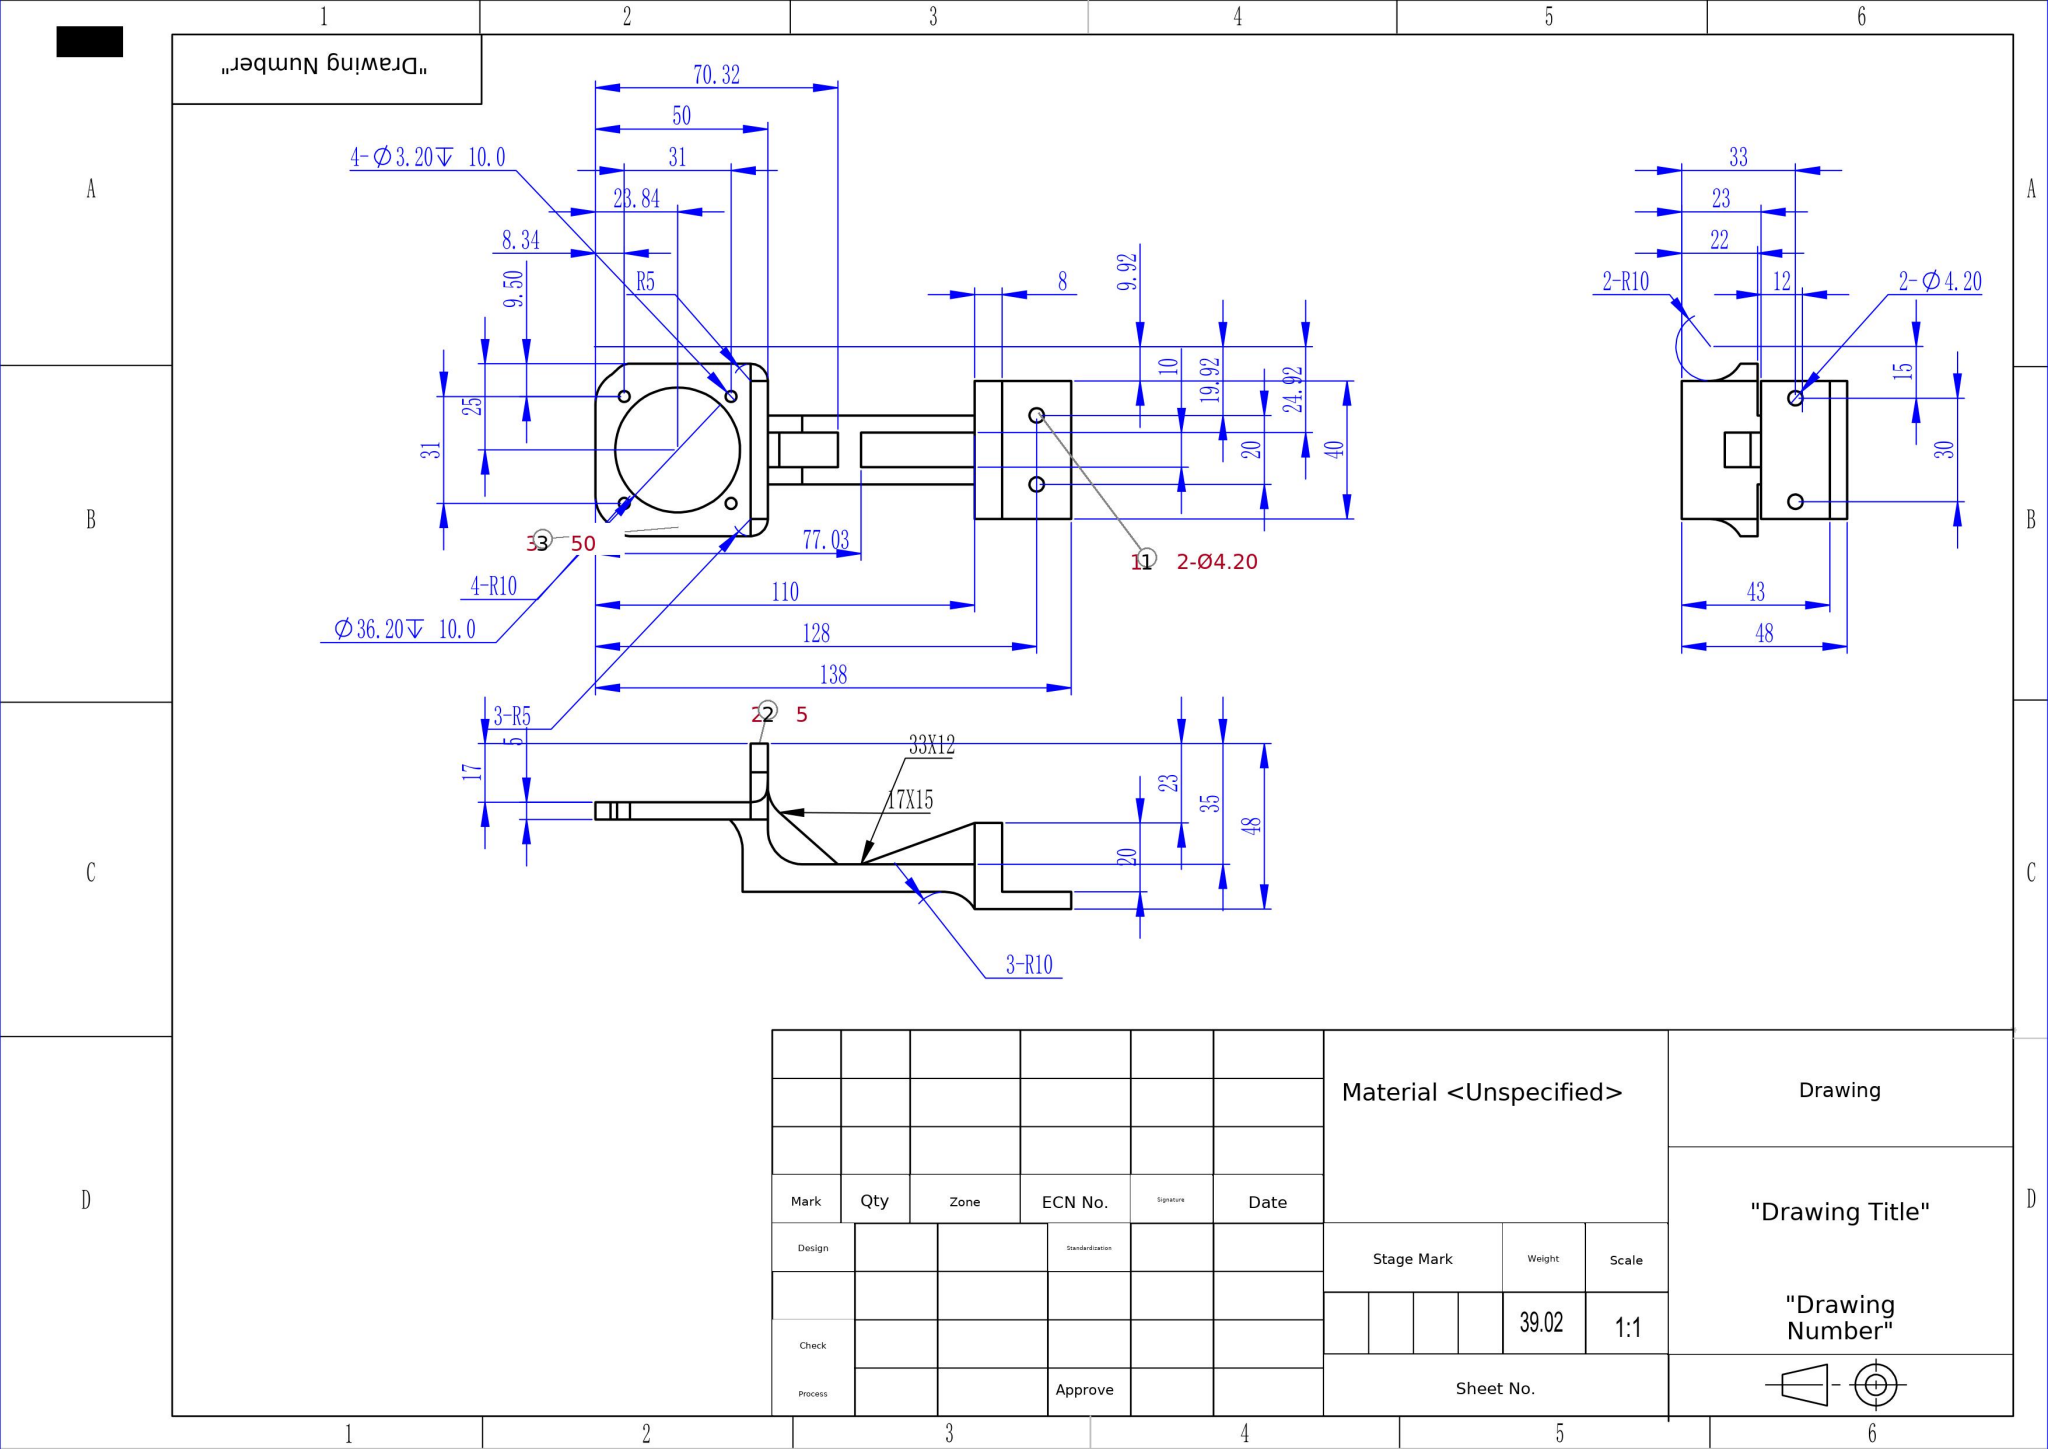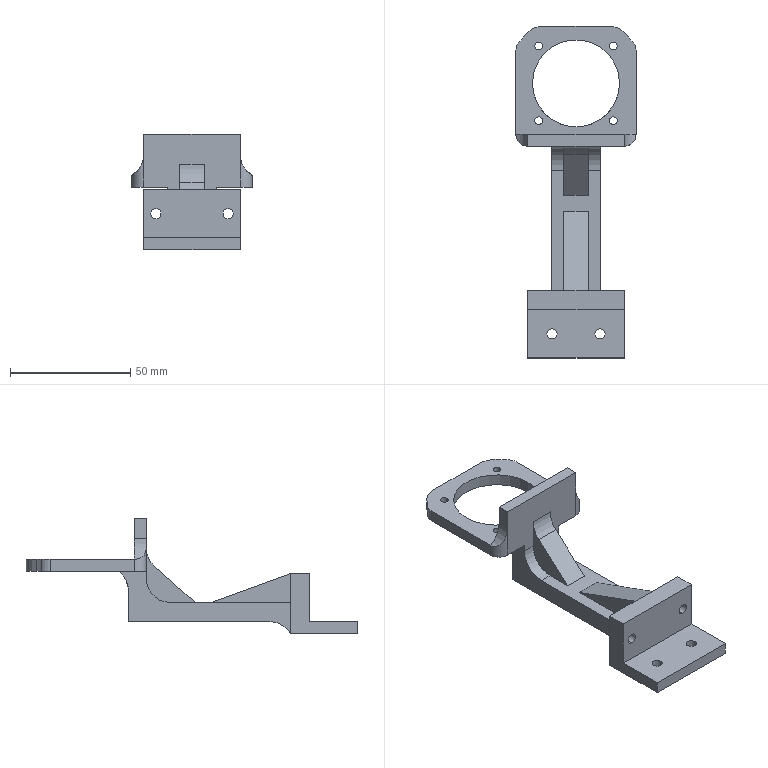Part | SolidWorks | mm | material <Unspecified> | 1 solid | 63 faces | box 50 x 138 x 48 mm | volume 39024 mm3 | cylinder 32 | plane 30 | spline 1 | commonest cylinder face diameters 20 x10 4.2 x8 3.2 x8 10 x4 36.2 x2